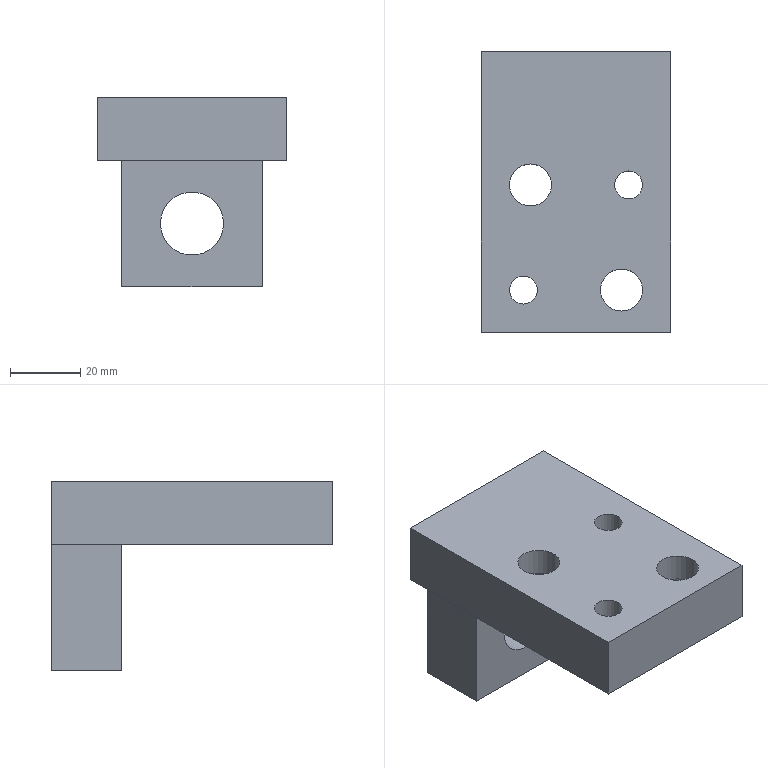Component | NX | SPACER_BLOCK | 1 solid | 19 faces | volume 92762 mm3 | plane 12 | cylinder 7 | commonest cylinder face diameters 18 x3 12 x2 8 x2